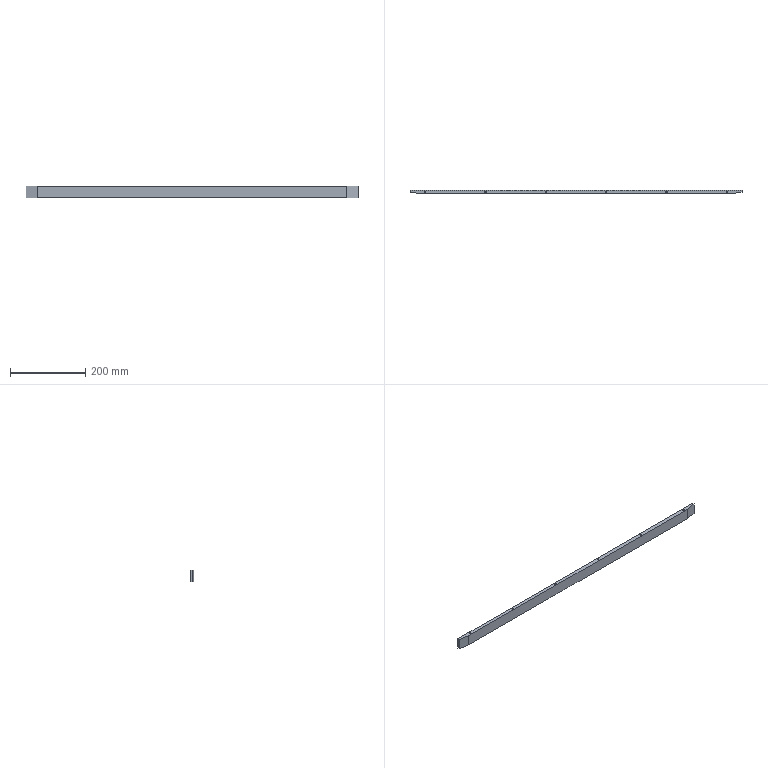Component | SolidWorks | --MA18S20041JR-SHuangGWSupportPlate2-1 | 1 solid | 56 faces | box 880 x 10 x 30 mm | volume 257369 mm3 | cylinder 24 | cone 24 | plane 8 | commonest cylinder face diameters 4.2 x24
build123d program:
from build123d import *
from OCP.BRepFilletAPI import BRepFilletAPI_MakeChamfer

# Parameters (mm, degrees)
SKETCH1_W             = 880
SKETCH1_H             = 30
EXTRUDE1_DEPTH        = 10
CHAMFER1_SIZE         = 5
CHAMFER1_SIZE2        = 30
M5_TAPPED_HOLE1_D     = 4.2
M5_TAPPED_HOLE1_DEPTH = 12.4
M5_TAPPED_HOLE1_TIP   = 1.262
M5_TAPPED_HOLE2_D     = 4.2
M5_TAPPED_HOLE2_DEPTH = 12.4
M5_TAPPED_HOLE2_TIP   = 1.262


with BuildPart() as part:
    # Sketch1 → Extrude1 (new body)
    with BuildSketch(Plane.XY):
        with Locations((440, -15)):
            Rectangle(SKETCH1_W, SKETCH1_H)
    extrude(amount=EXTRUDE1_DEPTH)

    # Chamfer1: one chamfer whose edges measure the first distance from different faces: ONE call of the kernel's chamfer builder (chamfer() names one face for all edges)
    chamfer1_edges_1 = [part.edges().sort_by_distance(p)[0] for p in [
        (880, -15, 10),
    ]]
    chamfer1_side_1 = [part.faces().sort_by_distance(p)[0] for p in [
        (880, -15, 5),
    ]]
    chamfer1_edges_2 = [part.edges().sort_by_distance(p)[0] for p in [
        (0, -15, 10),
    ]]
    chamfer1_side_2 = [part.faces().sort_by_distance(p)[0] for p in [
        (0, -15, 5),
    ]]
    chamfer1 = BRepFilletAPI_MakeChamfer(part.part.solid().wrapped)
    for e in chamfer1_edges_1:
        chamfer1.Add(CHAMFER1_SIZE, CHAMFER1_SIZE2, e.wrapped, chamfer1_side_1[0].wrapped)  # the first distance lies on this face
    for e in chamfer1_edges_2:
        chamfer1.Add(CHAMFER1_SIZE, CHAMFER1_SIZE2, e.wrapped, chamfer1_side_2[0].wrapped)  # the first distance lies on this face
    add(Compound.cast(chamfer1.Shape()), mode=Mode.REPLACE)

    # M5 Tapped Hole1
    with Locations(Plane(origin=(0, 0, 0), x_dir=(-1, 0, 0), z_dir=(0, 1, 0))):
        with Locations((-200, 5), (-40, 5), (-680, 5), (-840, 5), (-520, 5), (-360, 5)):
            Hole(M5_TAPPED_HOLE1_D / 2, depth=M5_TAPPED_HOLE1_DEPTH)
            with Locations((0, 0, -(M5_TAPPED_HOLE1_DEPTH + M5_TAPPED_HOLE1_TIP / 2))):  # 118° drill point
                Cone(0, M5_TAPPED_HOLE1_D / 2, M5_TAPPED_HOLE1_TIP, mode=Mode.SUBTRACT)

    # M5 Tapped Hole2
    with Locations(Plane.XZ.offset(30)):
        with Locations((40, 5), (200, 5), (680, 5), (840, 5), (360, 5), (520, 5)):
            Hole(M5_TAPPED_HOLE2_D / 2, depth=M5_TAPPED_HOLE2_DEPTH)
            with Locations((0, 0, -(M5_TAPPED_HOLE2_DEPTH + M5_TAPPED_HOLE2_TIP / 2))):  # 118° drill point
                Cone(0, M5_TAPPED_HOLE2_D / 2, M5_TAPPED_HOLE2_TIP, mode=Mode.SUBTRACT)


solid = part.part

# Placed as in the assembly
solid = solid.moved(Location((-142.956, 103.699, 49), (90, 0, 0)))